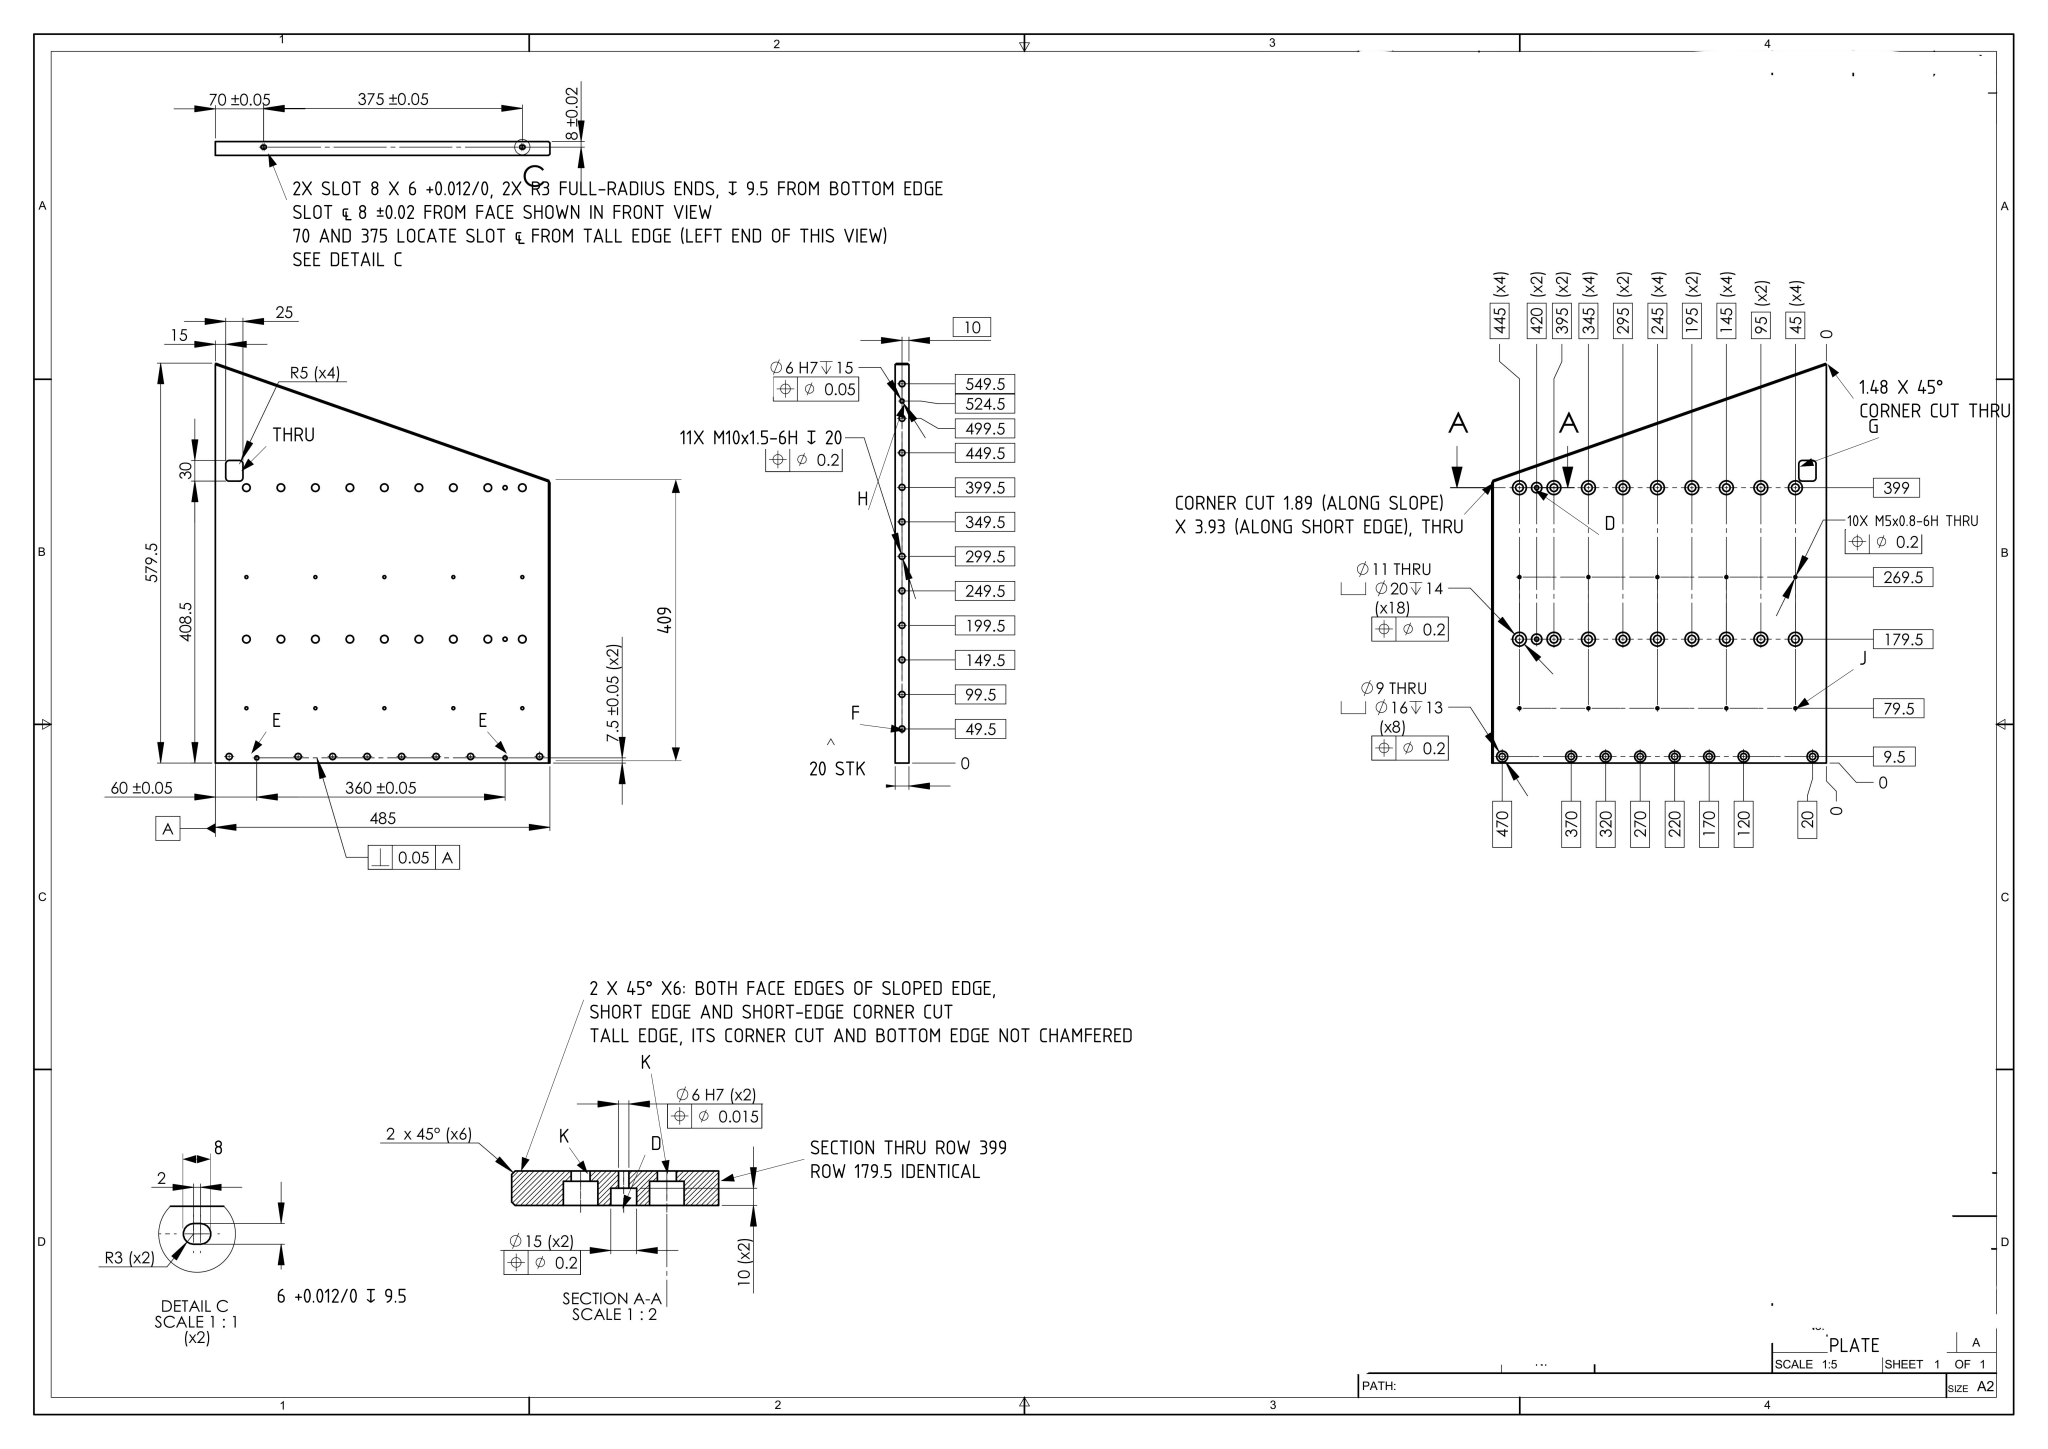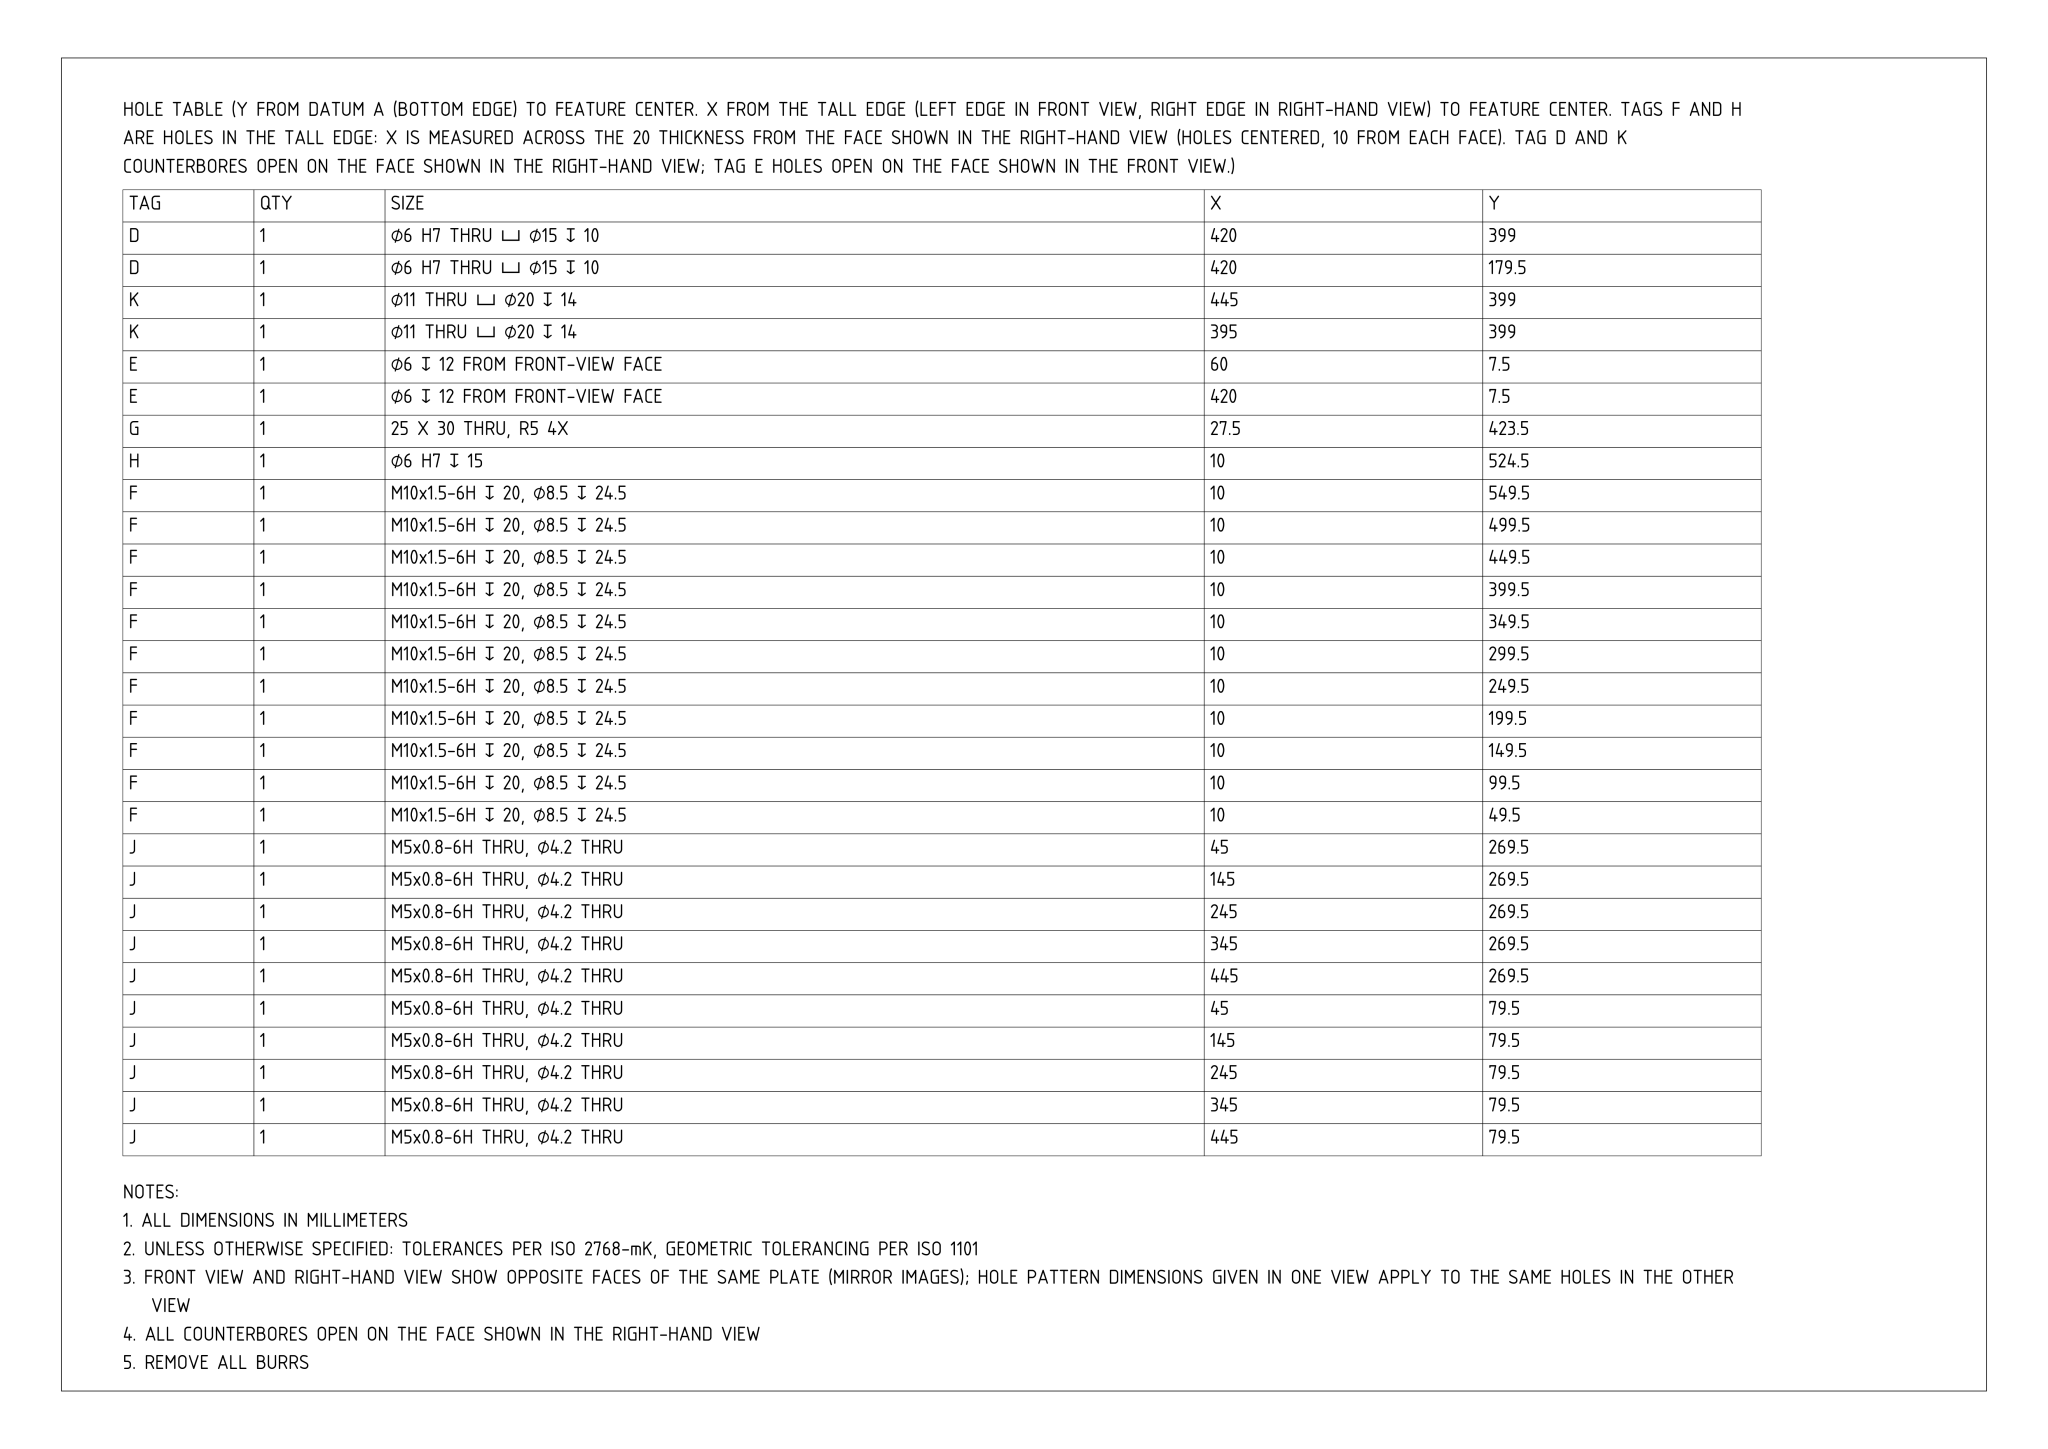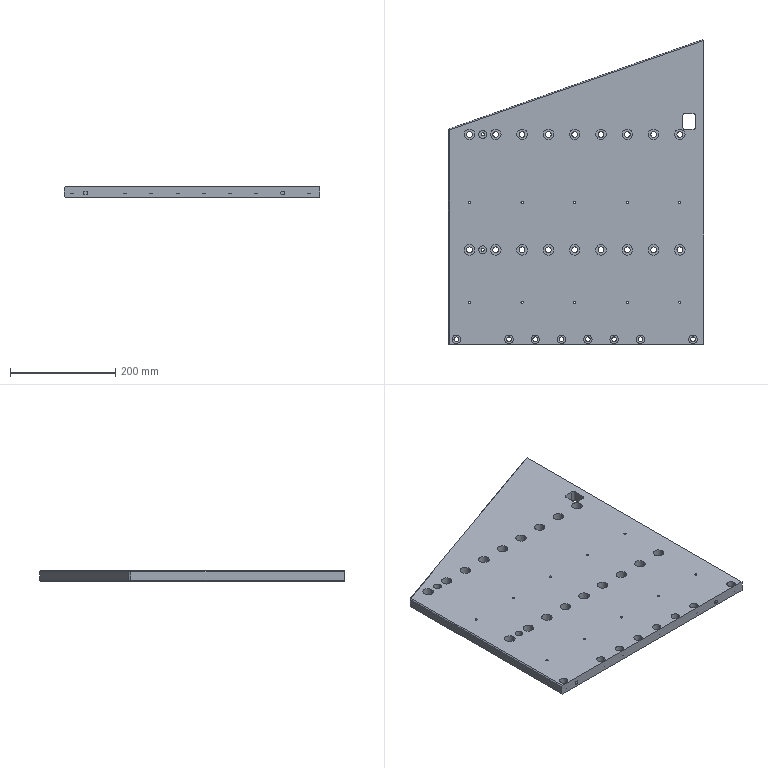Part | NX | mm | 1 solid | 248 faces | box 485 x 578.98 x 20 mm | volume 4637369 mm3 | cylinder 168 | plane 52 | cone 28 | commonest cylinder face diameters 11 x36 20 x36 8.5 x22 4.2 x20 9 x16 16 x16 6 x14 10 x4